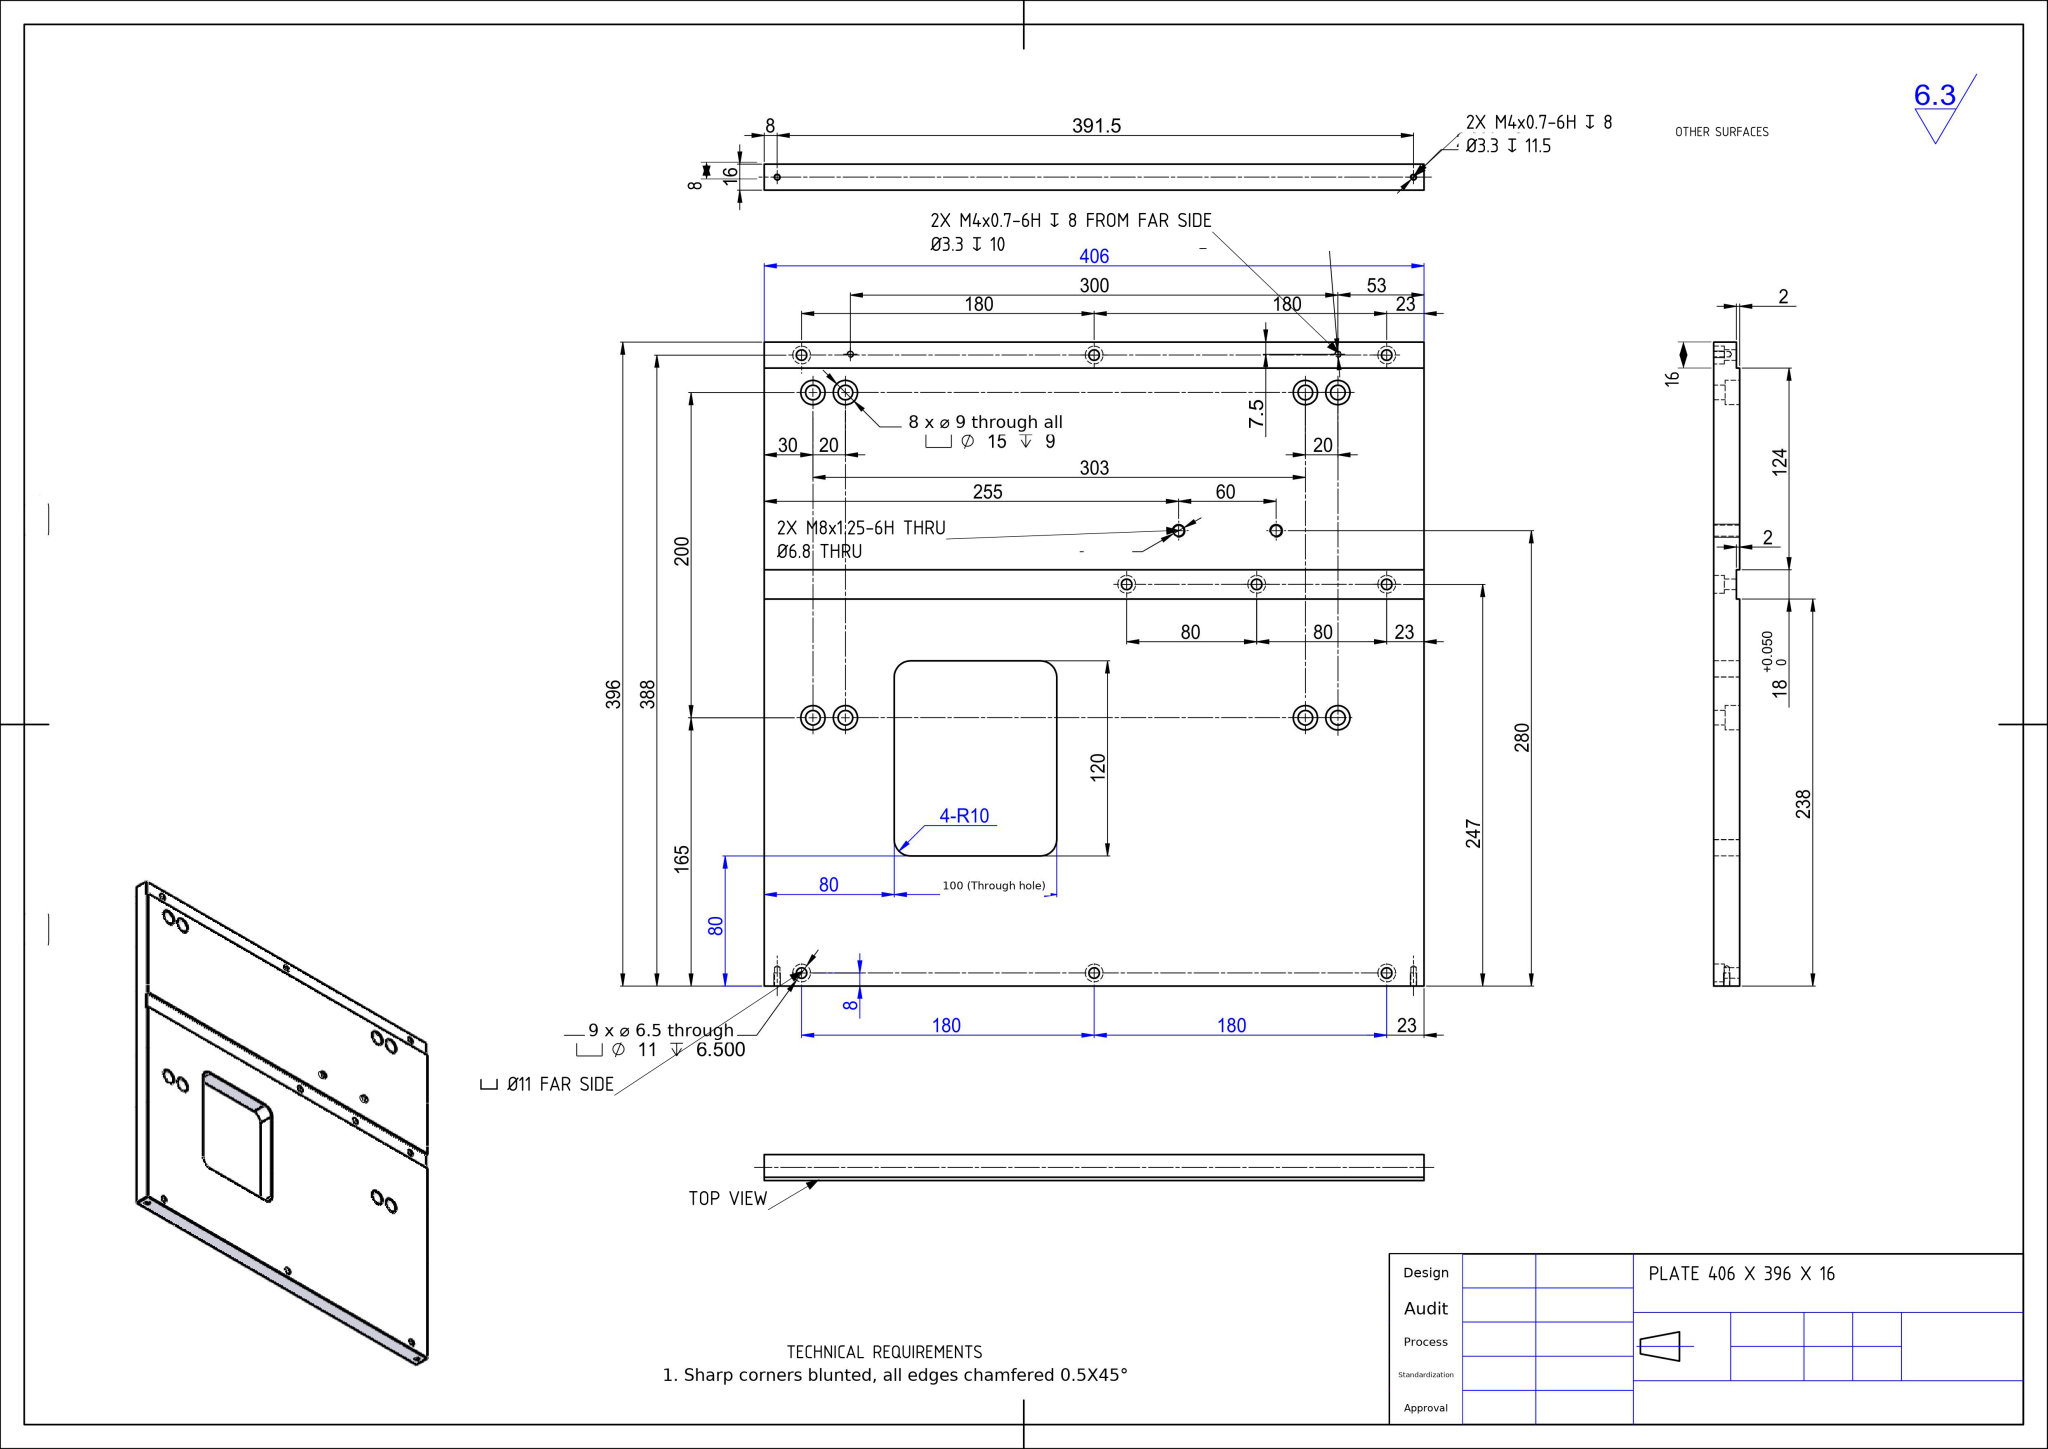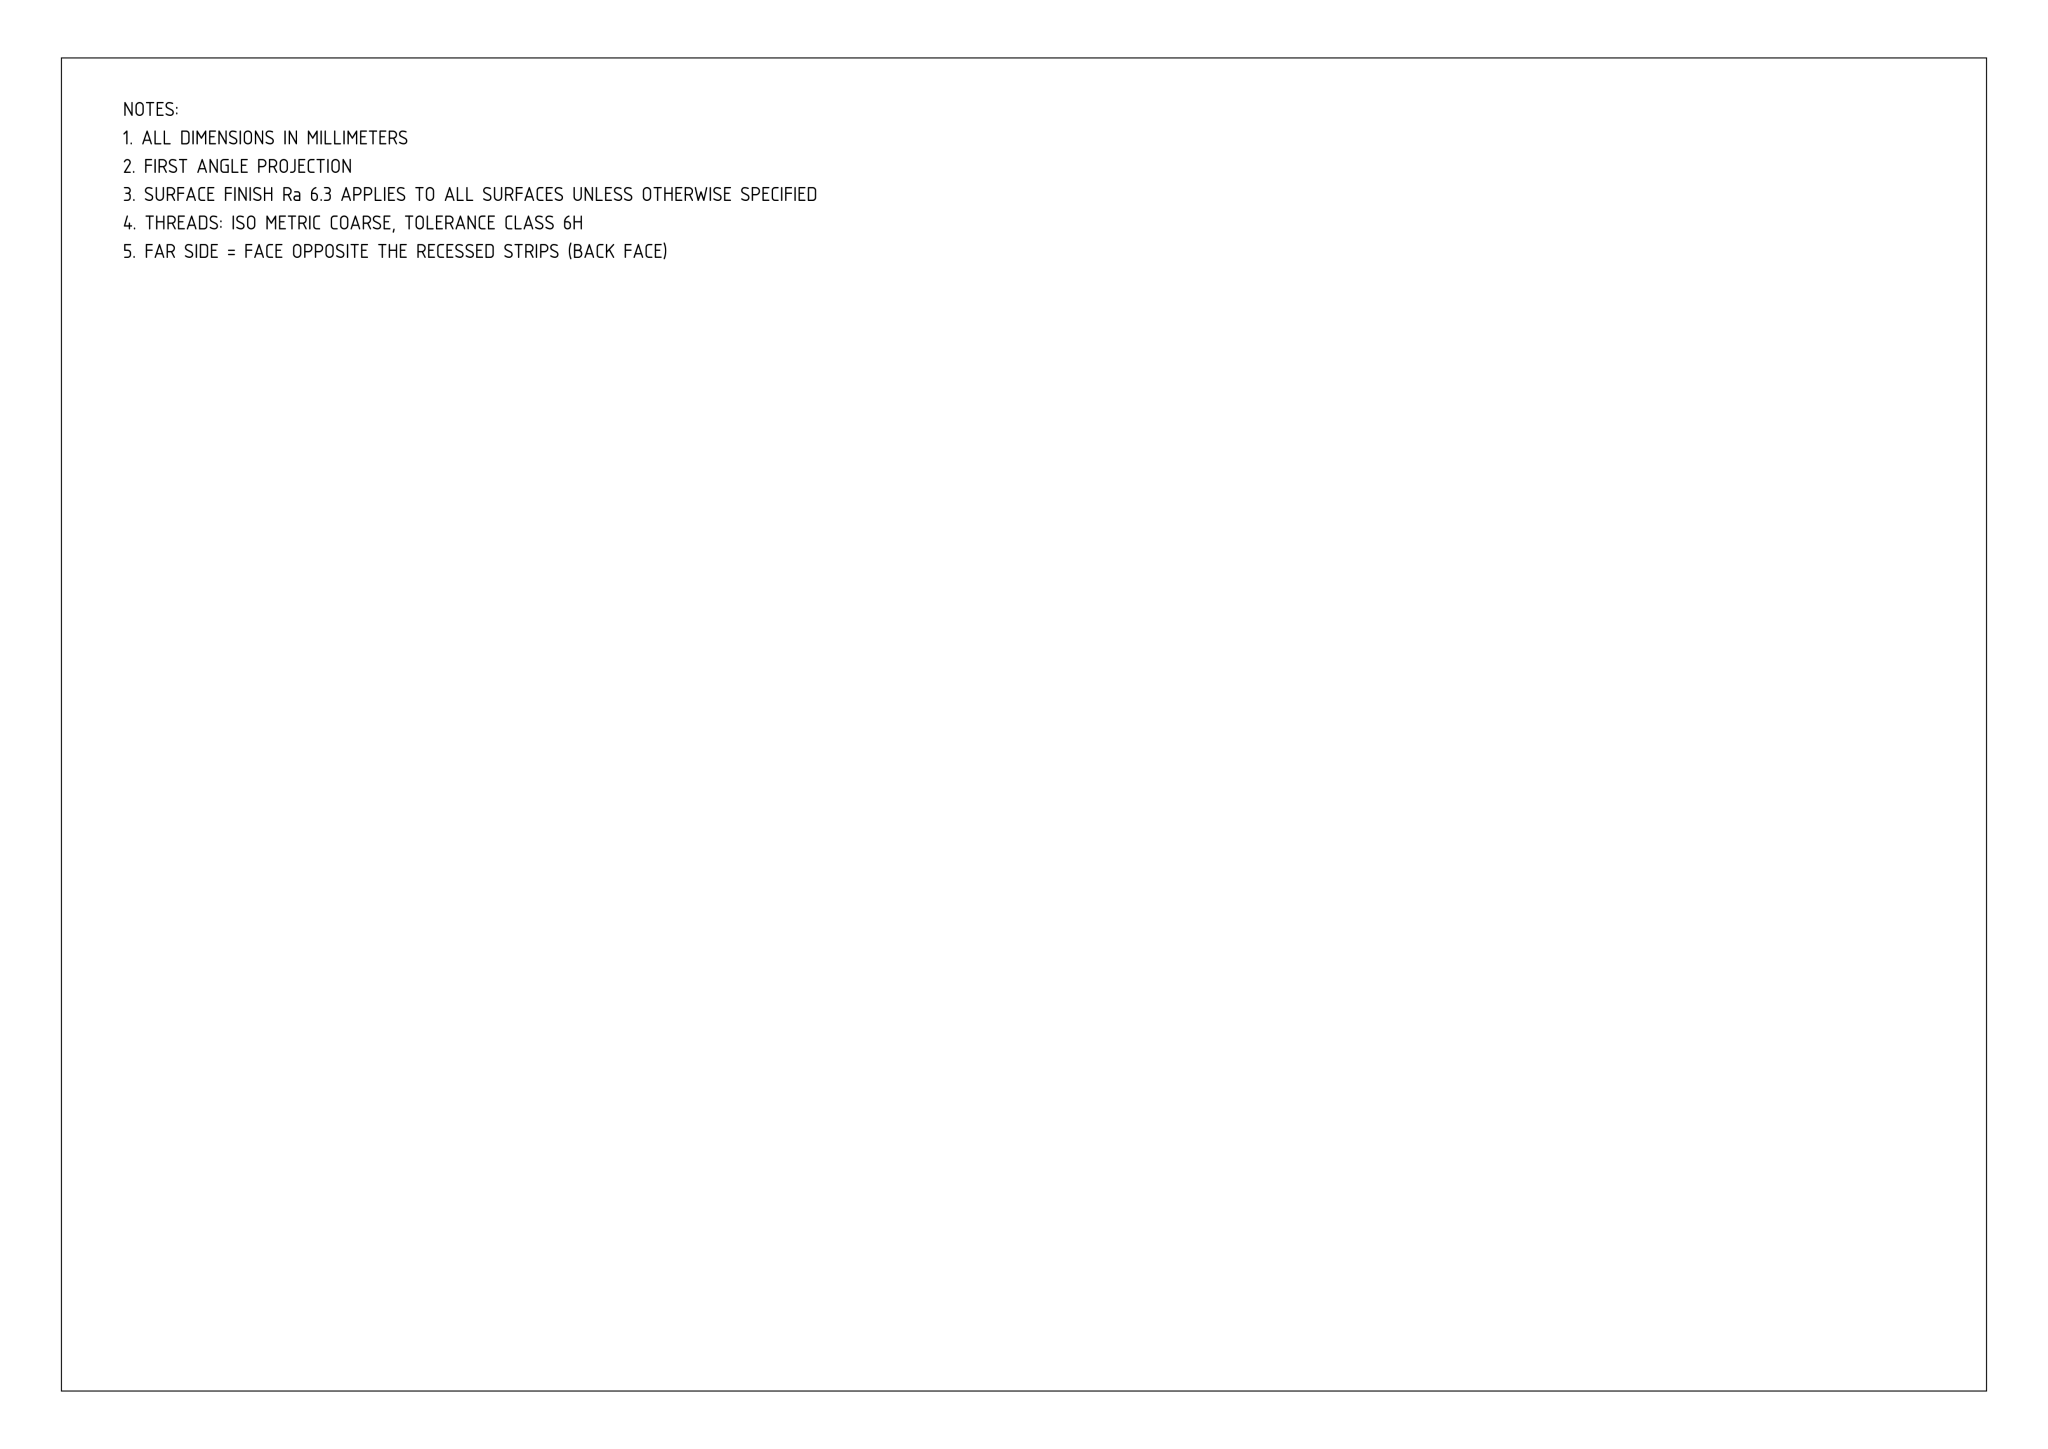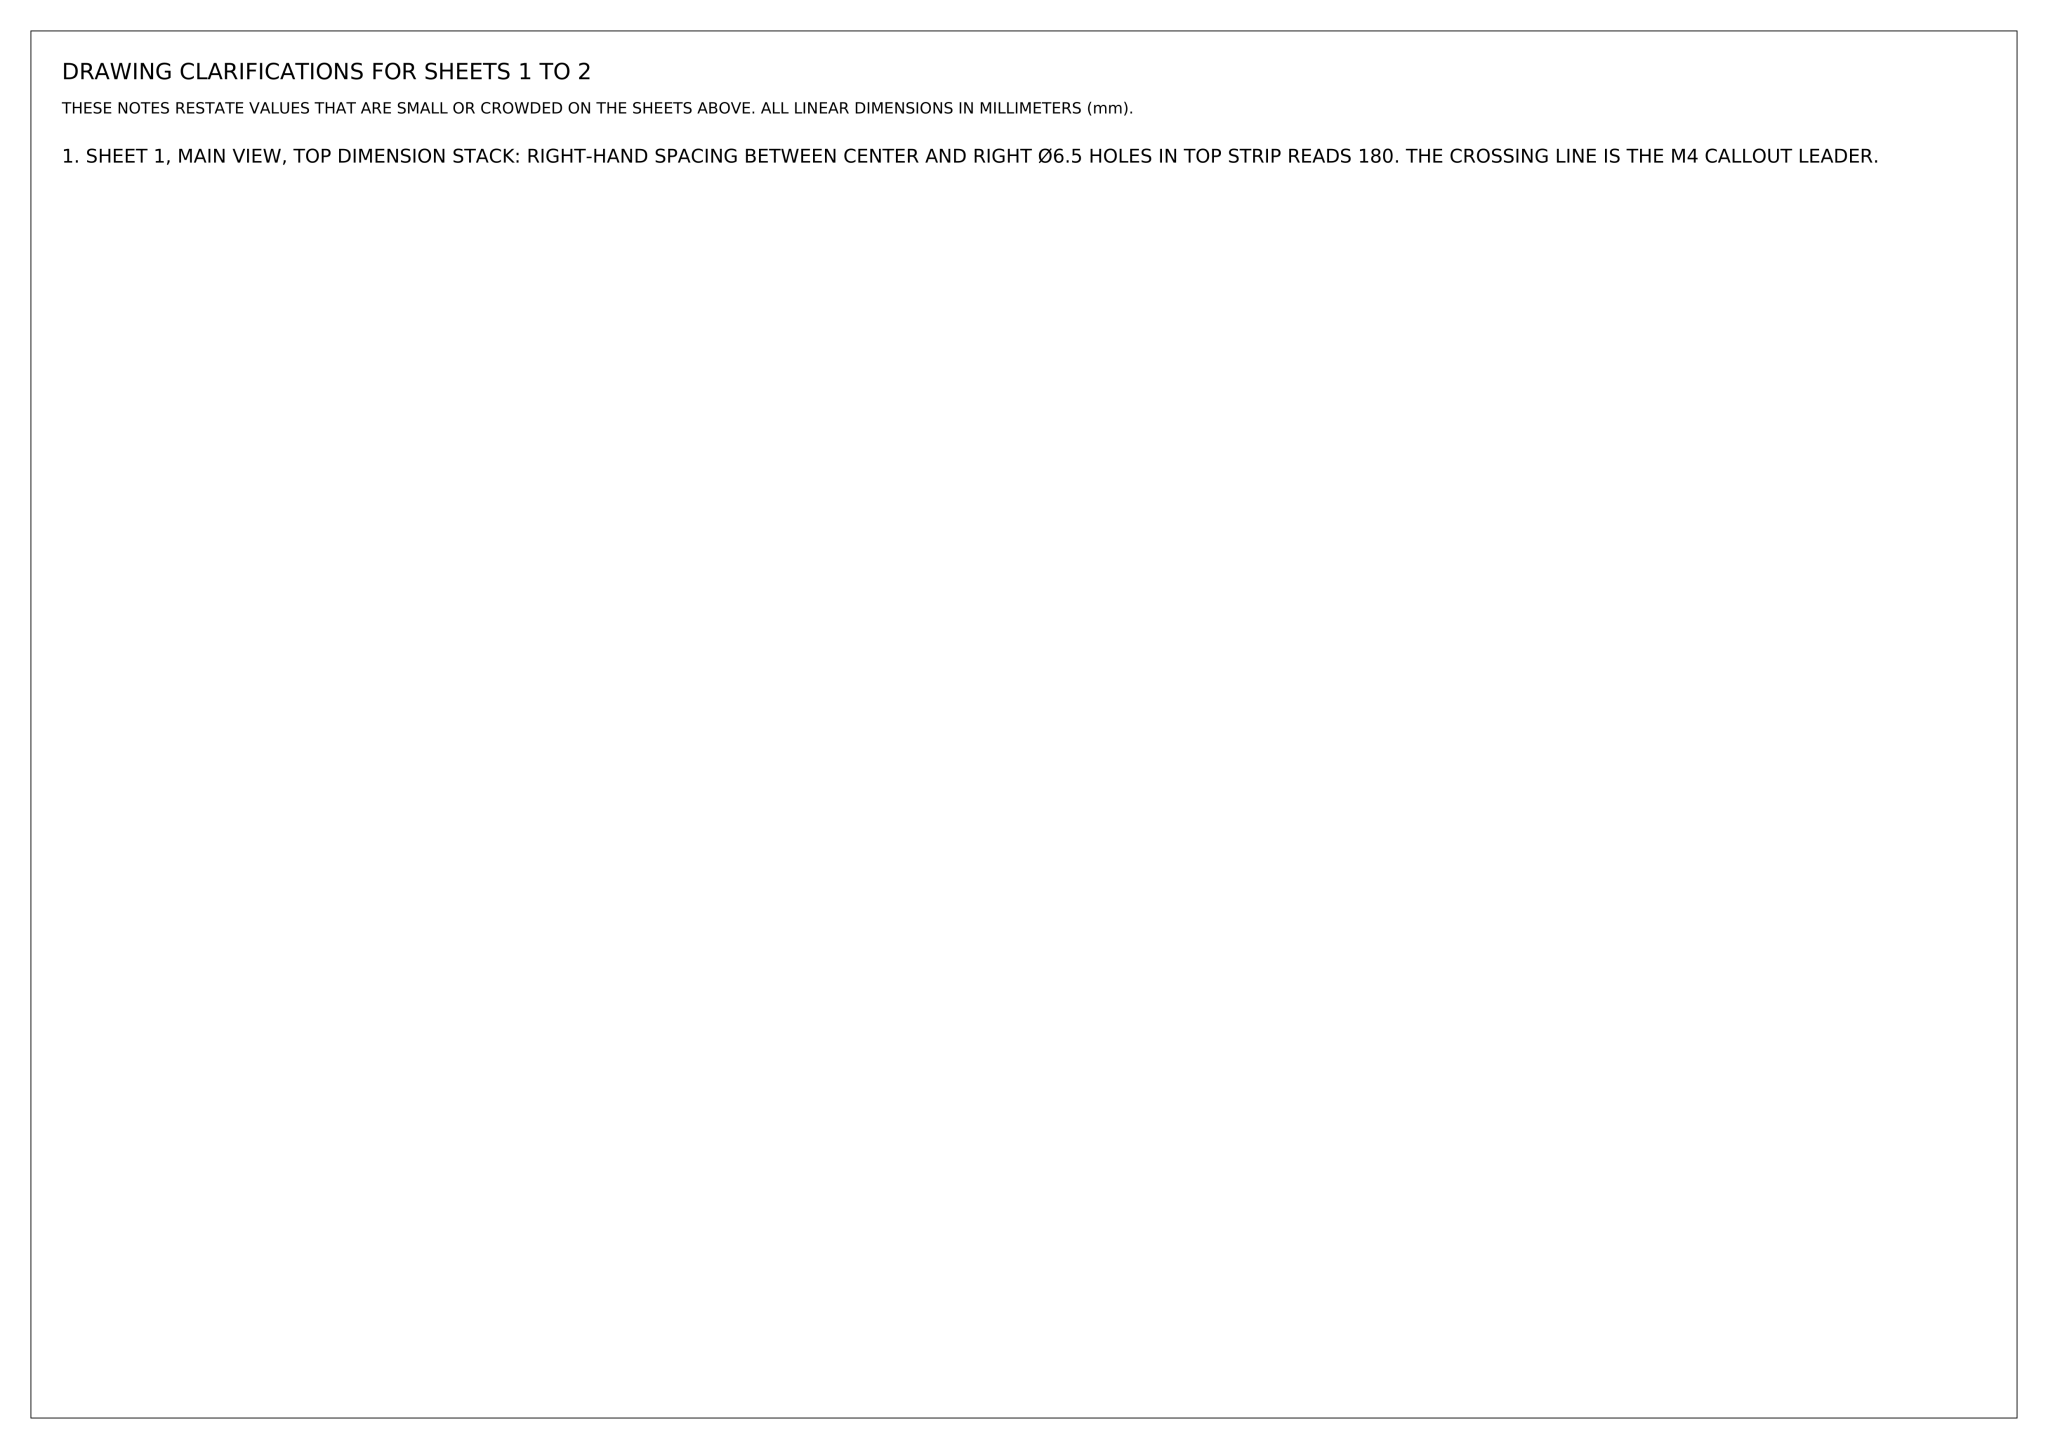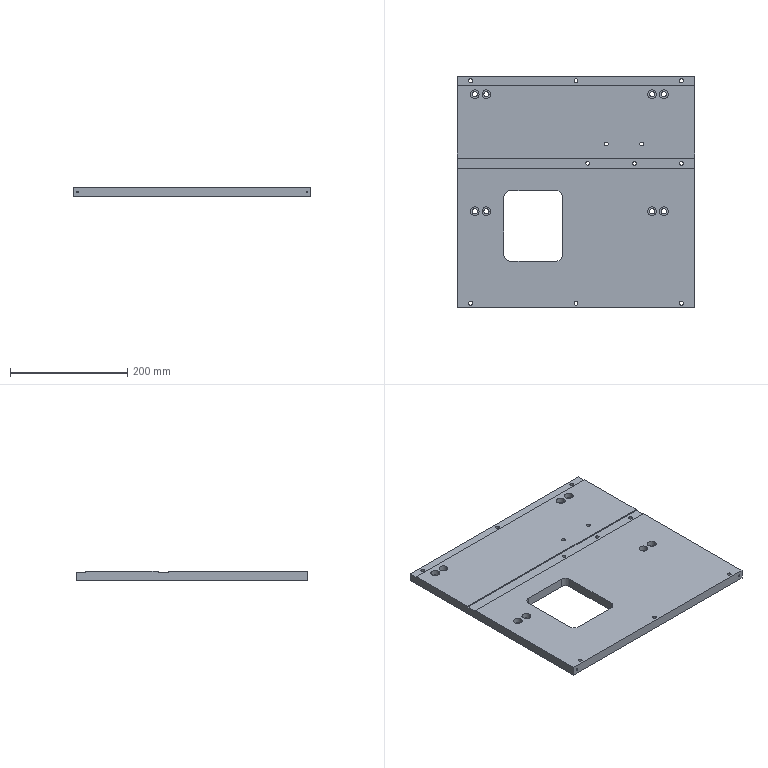Part | NX | mm | 1 solid | 125 faces | box 406 x 396 x 16 mm | volume 2328356 mm3 | cylinder 84 | plane 33 | cone 8 | commonest cylinder face diameters 11 x18 6.5 x18 9 x16 15 x16 3.3 x8 6.8 x4 20 x4